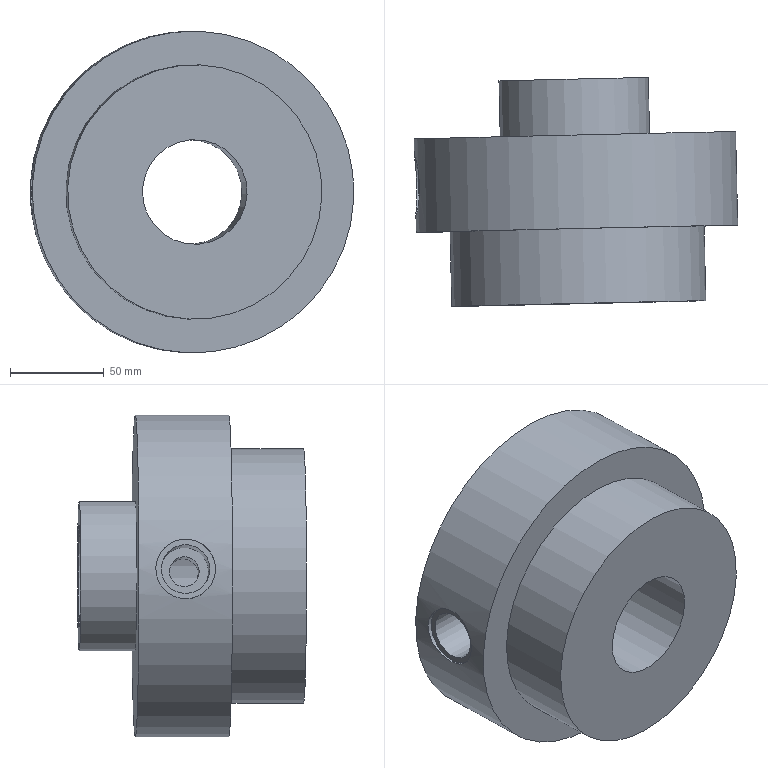Component | NX | 7 | 1 solid | 13 faces | volume 1574590 mm3 | cylinder 7 | plane 6 | commonest cylinder face diameters 56 x1 136 x1 172 x1 80 x1 32 x1 26 x1 16 x1